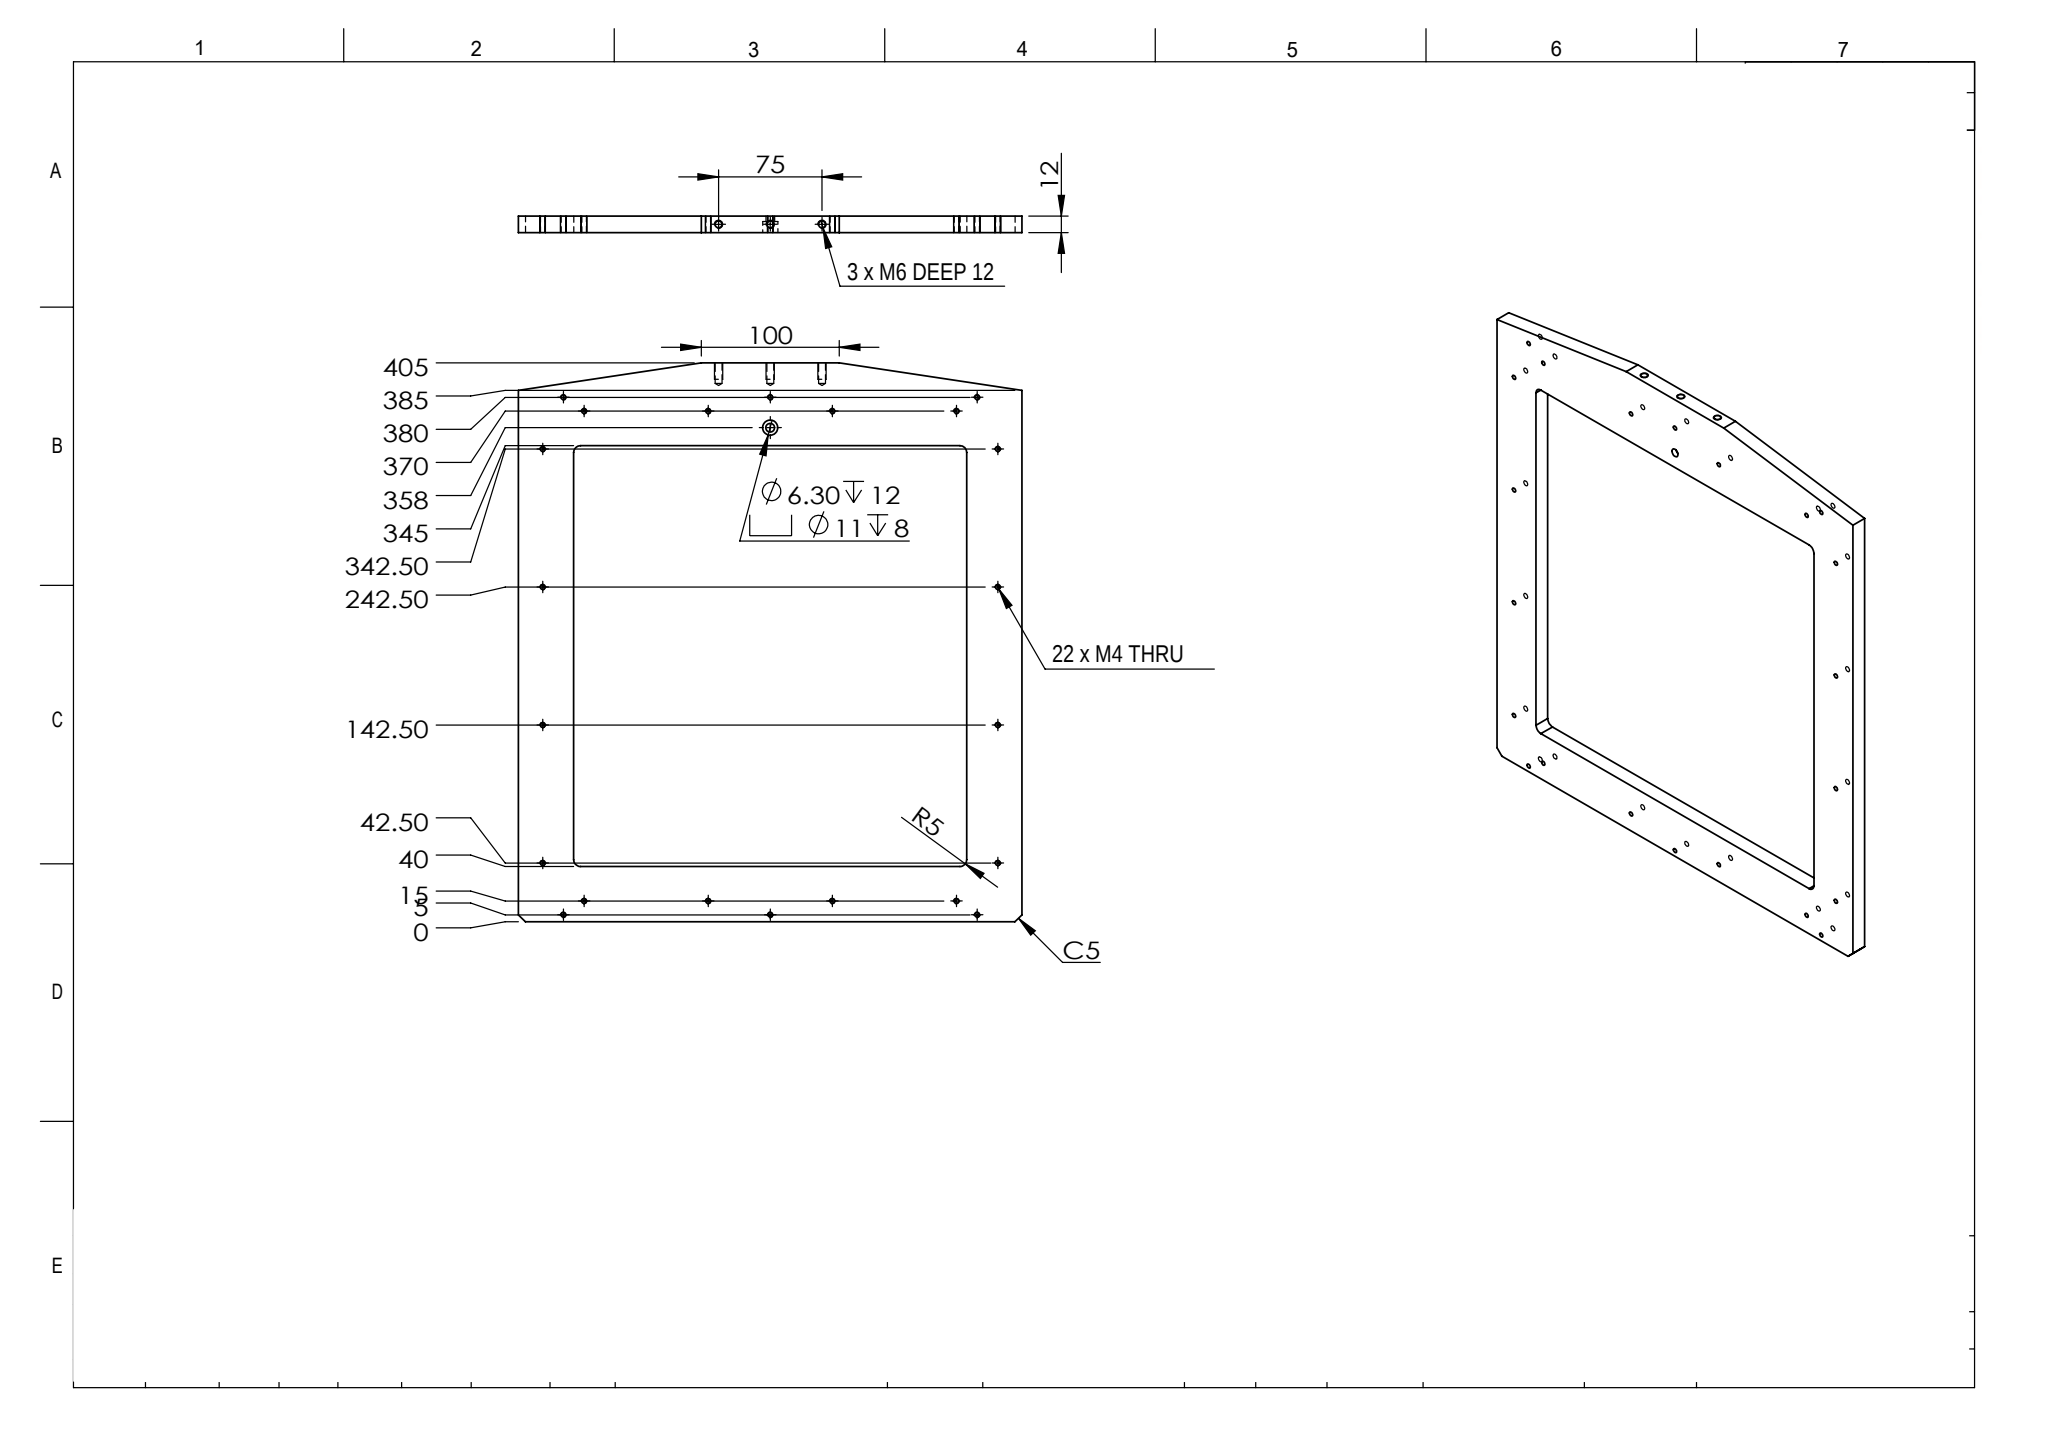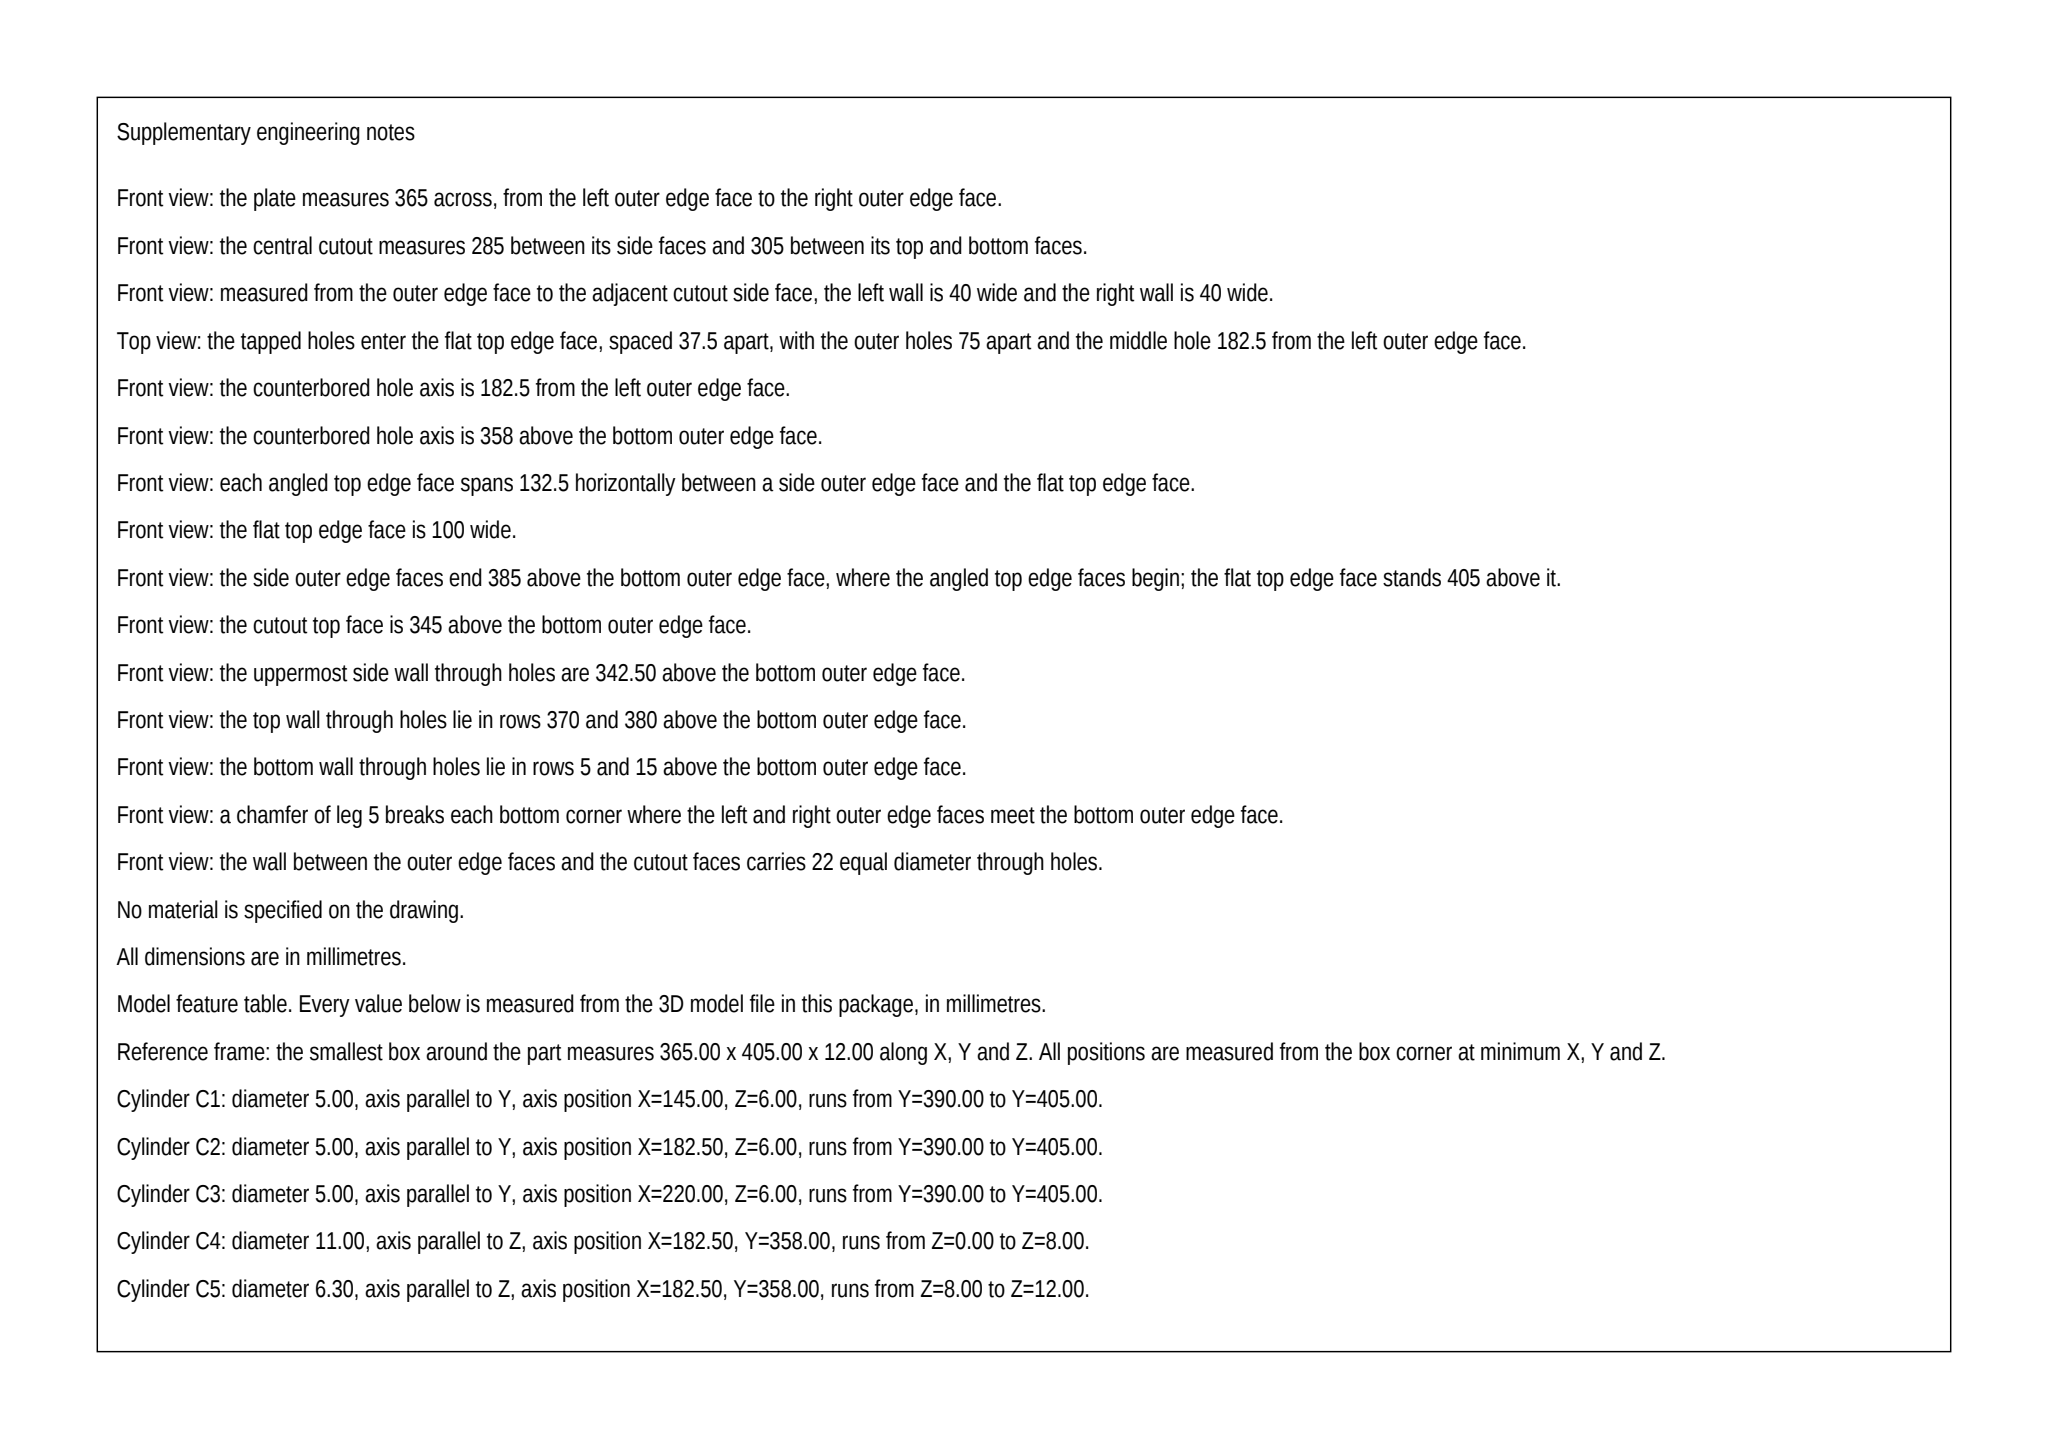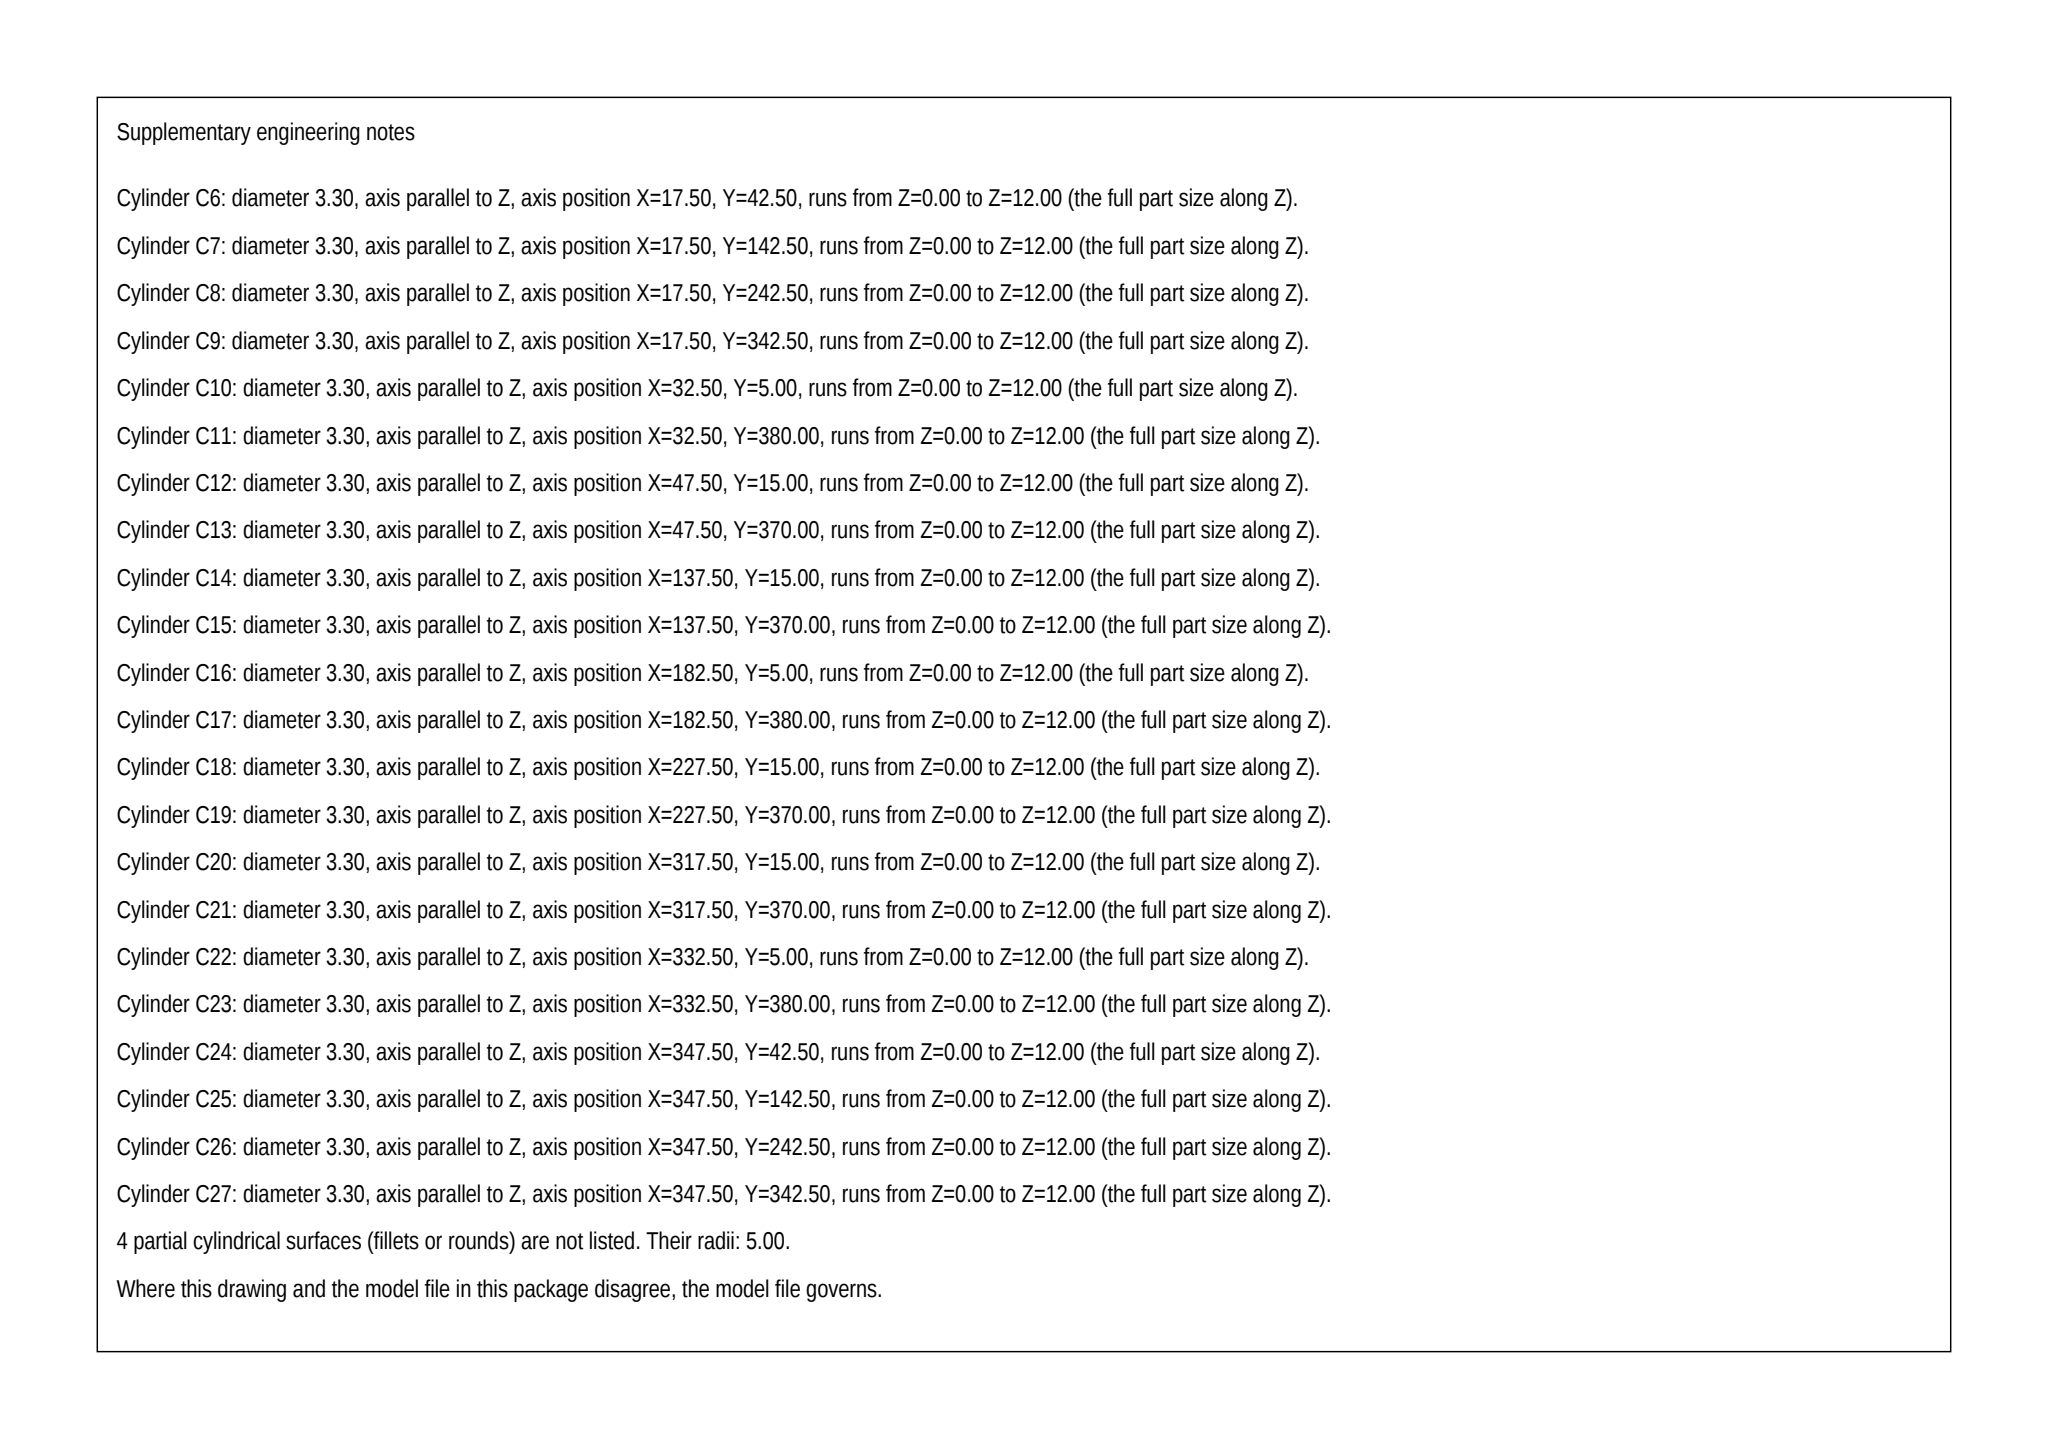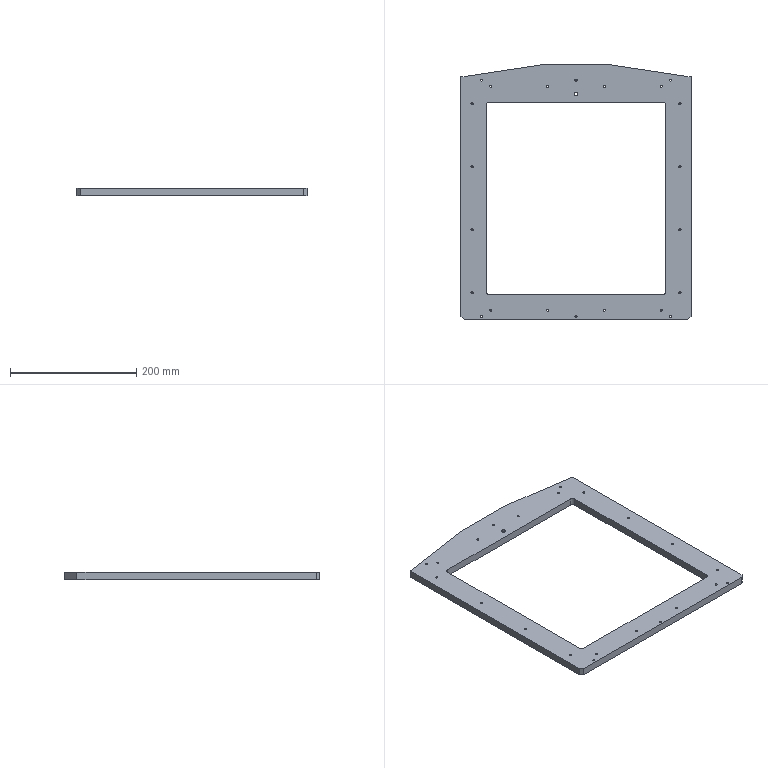Part | SolidWorks | mm | 1 solid | 79 faces | box 365 x 405 x 12 mm | volume 694902 mm3 | cylinder 58 | plane 15 | cone 6 | commonest cylinder face diameters 3.3 x44 5 x6 10 x4 11 x2 6.3 x2
build123d program:
from build123d import *

# Parameters (mm, degrees)
BOSS_EXTRUDE1_DEPTH   = 12
SKETCH2_W             = 285
SKETCH2_H             = 305
CUT_EXTRUDE1_DEPTH    = 281.369
M4_TAPPED_HOLE1_D     = 3.3
HOLE1_D               = 6.3
HOLE1_CBORE_D         = 11
HOLE1_CBORE_DEPTH     = 8
M6_TAPPED_HOLE1_D     = 5
M6_TAPPED_HOLE1_DEPTH = 15
M6_TAPPED_HOLE1_TIP   = 1.502
CHAMFER1_SIZE         = 5
FILLET1_R             = 5


with BuildPart() as part:
    # Sketch1 → Boss-Extrude1 (new body)
    with BuildSketch(Plane(origin=(0, 0, -6), x_dir=(-1, 0, 0), z_dir=(0, 0, -1))):
        Polygon((182.5, 192.5), (50, 212.5), (-50, 212.5), (-182.5, 192.5), (-182.5, -192.5), (182.5, -192.5), align=None)
    extrude(amount=-BOSS_EXTRUDE1_DEPTH)

    # Sketch2 → Cut-Extrude1 (cut, through all)
    with BuildSketch(Plane.XY.offset(6)):
        Rectangle(SKETCH2_W, SKETCH2_H)
    extrude(amount=-CUT_EXTRUDE1_DEPTH, mode=Mode.SUBTRACT)

    # M4 Tapped Hole1 (through all)
    with Locations(Plane(origin=(0, 0, -6), x_dir=(-1, 0, 0), z_dir=(0, 0, -1))):
        with Locations((135, -177.5), (45, -177.5), (-45, -177.5), (-135, -177.5), (165, -150), (165, -50), (165, 50), (165, 150), (-165, -150), (-165, -50), (-165, 50), (-165, 150), (-135, 177.5), (-45, 177.5), (45, 177.5), (135, 177.5), (150, 187.5), (-150, 187.5), (-150, -187.5), (150, -187.5), (0, 187.5), (0, -187.5)):
            Hole(M4_TAPPED_HOLE1_D / 2)

    # Hole1 (through all)
    with Locations(Plane(origin=(0, 0, -6), x_dir=(-1, 0, 0), z_dir=(0, 0, -1))):
        with Locations((0, 165.5)):
            CounterBoreHole(HOLE1_D / 2, HOLE1_CBORE_D / 2, HOLE1_CBORE_DEPTH)

    # M6 Tapped Hole1
    with Locations(Plane(origin=(0, 212.5, 0), x_dir=(1, 0, 0), z_dir=(0, 1, 0))):
        with Locations((37.5, 0), (0, 0), (-37.5, 0)):
            Hole(M6_TAPPED_HOLE1_D / 2, depth=M6_TAPPED_HOLE1_DEPTH)
            with Locations((0, 0, -(M6_TAPPED_HOLE1_DEPTH + M6_TAPPED_HOLE1_TIP / 2))):  # 118° drill point
                Cone(0, M6_TAPPED_HOLE1_D / 2, M6_TAPPED_HOLE1_TIP, mode=Mode.SUBTRACT)

    # Chamfer1
    chamfer1_edges = [part.edges().sort_by_distance(p)[0] for p in [
        (-182.5, -192.5, 0),
        (182.5, -192.5, 0),
    ]]
    chamfer(chamfer1_edges, length=CHAMFER1_SIZE)

    # Fillet1
    fillet1_edges = [part.edges().sort_by_distance(p)[0] for p in [
        (-142.5, -152.5, 0),
        (-142.5, 152.5, 0),
        (142.5, 152.5, 0),
        (142.5, -152.5, 0),
    ]]
    fillet(fillet1_edges, radius=FILLET1_R)


solid = part.part